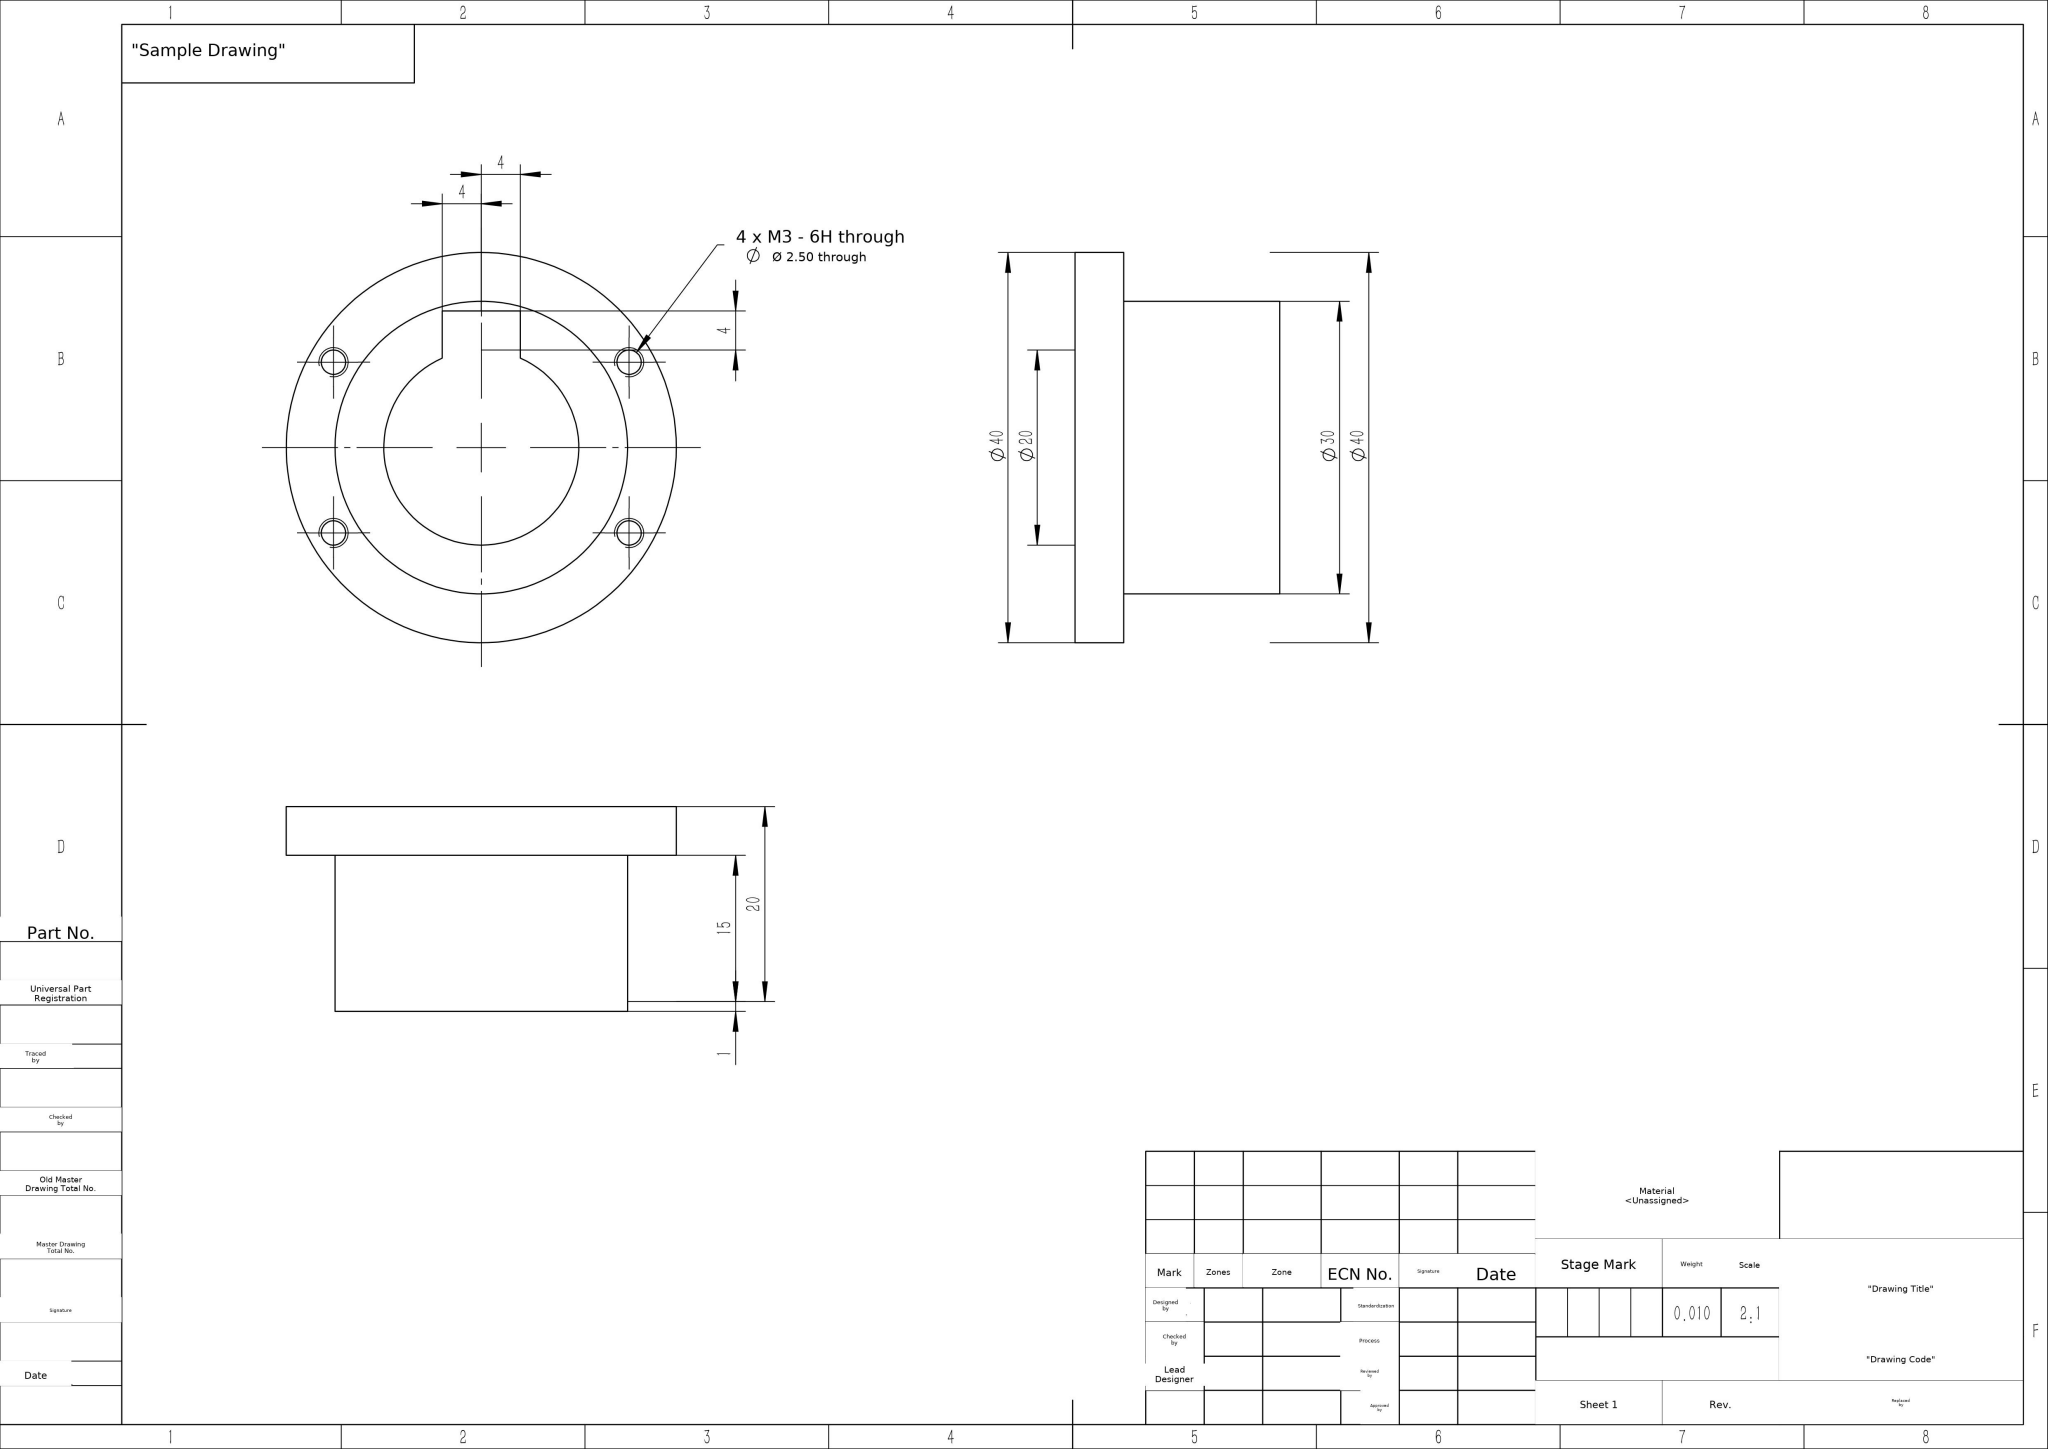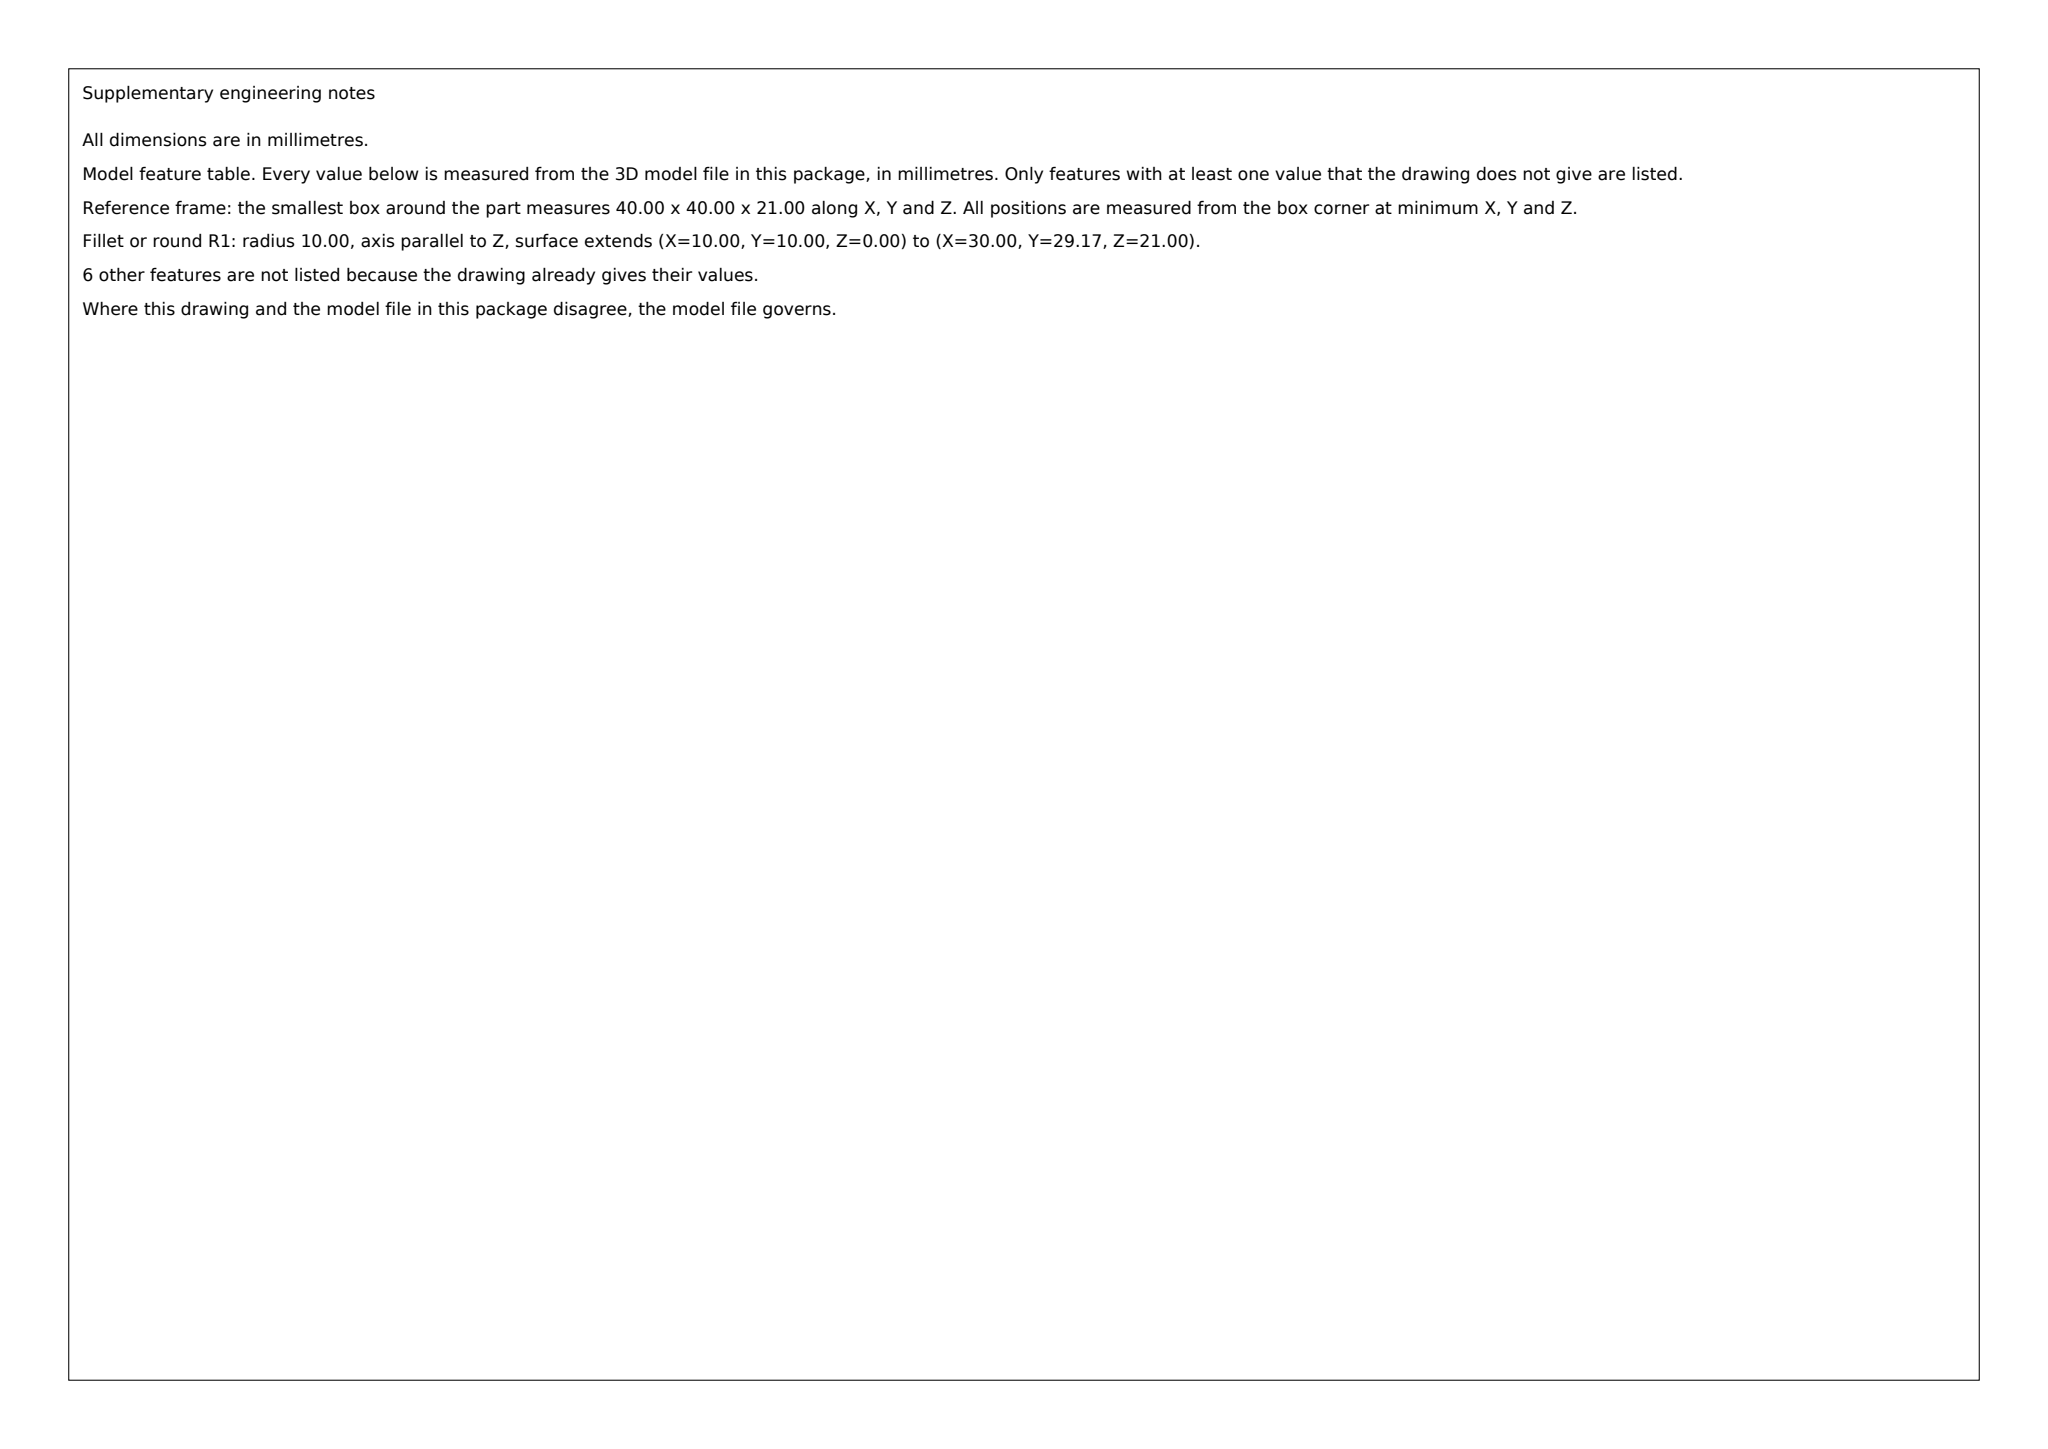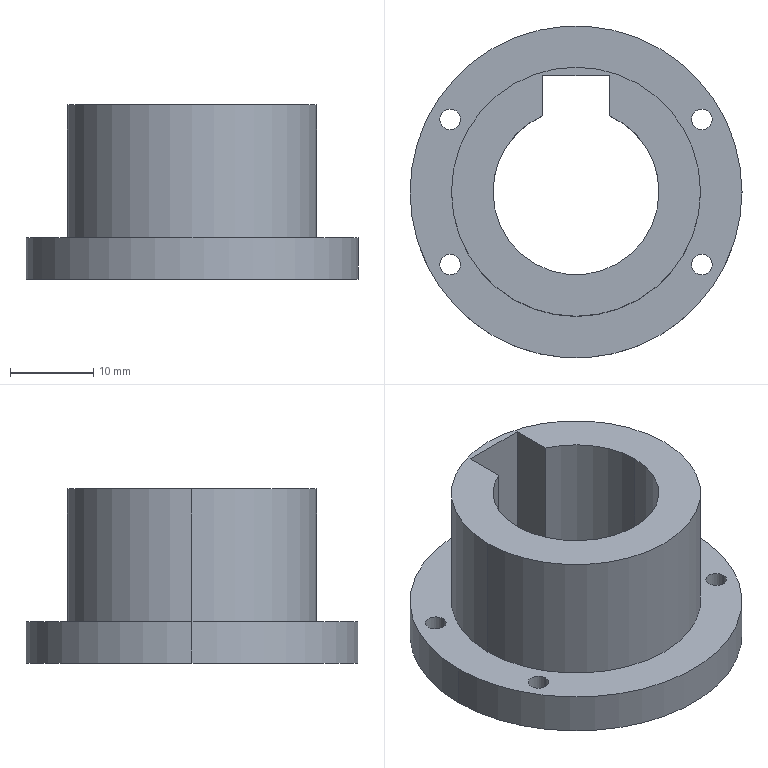Part | SolidWorks | mm | 1 solid | 21 faces | box 40 x 40 x 21 mm | volume 10179 mm3 | cylinder 15 | plane 6 | commonest cylinder face diameters 2.5 x8 20 x3 30 x2 40 x2
build123d program:
from build123d import *

# Parameters (mm, degrees)
SKETCH1_R           = 20
SKETCH1_R_2         = 10
BOSS_EXTRUDE1_DEPTH = 20
CUT_EXTRUDE1_START  = -20
CUT_EXTRUDE1_DEPTH  = 20
CUT_EXTRUDE3_START  = -15
SKETCH4_R           = 20
SKETCH4_R_2         = 15
CUT_EXTRUDE3_DEPTH  = 15
M3_TAPPED_HOLE1_D   = 2.5
SKETCH7_R           = 15
BOSS_EXTRUDE2_DEPTH = 1


with BuildPart() as part:
    # Sketch1 → Boss-Extrude1 (new body)
    with BuildSketch(Plane.XY):
        Circle(SKETCH1_R)
        Circle(SKETCH1_R_2, mode=Mode.SUBTRACT)
    extrude(amount=BOSS_EXTRUDE1_DEPTH)

    # Sketch3 → Cut-Extrude1 (cut)
    with BuildSketch(Plane.XY.offset(20).offset(CUT_EXTRUDE1_START)):
        with BuildLine():
            ThreePointArc((-4, 9.165), (-2.043, 9.789), (0, 10))
            Line((0, 10), (0, 14))
            Line((0, 14), (-4, 14))
            Line((-4, 14), (-4, 9.165))
        make_face()
        with BuildLine():
            Line((0, 14), (0, 10))
            ThreePointArc((0, 10), (2.043, 9.789), (4, 9.165))
            Line((4, 9.165), (4, 14))
            Line((4, 14), (0, 14))
        make_face()
    extrude(amount=CUT_EXTRUDE1_DEPTH, mode=Mode.SUBTRACT)

    # Sketch4 → Cut-Extrude3 (cut)
    with BuildSketch(Plane.XY.offset(20).offset(CUT_EXTRUDE3_START)):
        Circle(SKETCH4_R)
        Circle(SKETCH4_R_2, mode=Mode.SUBTRACT)
    extrude(amount=CUT_EXTRUDE3_DEPTH, mode=Mode.SUBTRACT)

    # M3 Tapped Hole1 (through all)
    with Locations(Plane(origin=(15.155, 8.75, 0), x_dir=(-1, 0, 0), z_dir=(0, 0, -1))):
        with Locations((0, 0), (30.311, 0), (30.311, -17.5), (0, -17.5)):
            Hole(M3_TAPPED_HOLE1_D / 2)

    # Sketch7 → Boss-Extrude2 (add)
    with BuildSketch(Plane.XY.offset(20)):
        Circle(SKETCH7_R)
        with BuildLine():
            Line((-4, 9.165), (-4, 14))
            Line((-4, 14), (4, 14))
            Line((4, 14), (4, 9.165))
            ThreePointArc((4, 9.165), (0, -10), (-4, 9.165))
        make_face(mode=Mode.SUBTRACT)
    extrude(amount=BOSS_EXTRUDE2_DEPTH)


solid = part.part
STEP:
#1=CARTESIAN_POINT('',(13.905,8.75,5.));
#2=VERTEX_POINT('',#1);
#3=CARTESIAN_POINT('',(16.405,8.75,5.));
#4=VERTEX_POINT('',#3);
#5=CARTESIAN_POINT('',(15.155,8.75,5.));
#6=DIRECTION('',(0.,0.,1.));
#7=DIRECTION('',(1.,0.,0.));
#8=AXIS2_PLACEMENT_3D('',#5,#6,#7);
#9=CIRCLE('',#8,1.25);
#10=EDGE_CURVE('',#2,#4,#9,.T.);
#11=ORIENTED_EDGE('',*,*,#10,.T.);
#12=CARTESIAN_POINT('',(16.405,8.75,-0.));
#13=VERTEX_POINT('',#12);
#14=CARTESIAN_POINT('',(16.405,8.75,0.));
#15=DIRECTION('',(0.,0.,-1.));
#16=VECTOR('',#15,1000.);
#17=LINE('',#14,#16);
#18=EDGE_CURVE('',#4,#13,#17,.T.);
#19=ORIENTED_EDGE('',*,*,#18,.T.);
#20=CARTESIAN_POINT('',(13.905,8.75,-0.));
#21=VERTEX_POINT('',#20);
#22=CARTESIAN_POINT('',(15.155,8.75,-0.));
#23=DIRECTION('',(0.,0.,-1.));
#24=DIRECTION('',(-1.,0.,0.));
#25=AXIS2_PLACEMENT_3D('',#22,#23,#24);
#26=CIRCLE('',#25,1.25);
#27=EDGE_CURVE('',#13,#21,#26,.T.);
#28=ORIENTED_EDGE('',*,*,#27,.T.);
#29=CARTESIAN_POINT('',(13.905,8.75,0.));
#30=DIRECTION('',(0.,0.,-1.));
#31=VECTOR('',#30,1000.);
#32=LINE('',#29,#31);
#33=EDGE_CURVE('',#2,#21,#32,.T.);
#34=ORIENTED_EDGE('',*,*,#33,.F.);
#35=EDGE_LOOP('',(#11,#19,#28,#34));
#36=FACE_OUTER_BOUND('',#35,.T.);
#37=CARTESIAN_POINT('',(15.155,8.75,0.));
#38=DIRECTION('',(0.,0.,-1.));
#39=DIRECTION('',(-1.,0.,0.));
#40=AXIS2_PLACEMENT_3D('',#37,#38,#39);
#41=CYLINDRICAL_SURFACE('',#40,1.25);
#42=ADVANCED_FACE('',(#36),#41,.F.);
#43=CARTESIAN_POINT('',(-16.405,8.75,5.));
#44=VERTEX_POINT('',#43);
#45=CARTESIAN_POINT('',(-13.905,8.75,5.));
#46=VERTEX_POINT('',#45);
#47=CARTESIAN_POINT('',(-15.155,8.75,5.));
#48=DIRECTION('',(0.,0.,1.));
#49=DIRECTION('',(1.,0.,0.));
#50=AXIS2_PLACEMENT_3D('',#47,#48,#49);
#51=CIRCLE('',#50,1.25);
#52=EDGE_CURVE('',#44,#46,#51,.T.);
#53=ORIENTED_EDGE('',*,*,#52,.T.);
#54=CARTESIAN_POINT('',(-13.905,8.75,-0.));
#55=VERTEX_POINT('',#54);
#56=CARTESIAN_POINT('',(-13.905,8.75,0.));
#57=DIRECTION('',(0.,0.,-1.));
#58=VECTOR('',#57,1000.);
#59=LINE('',#56,#58);
#60=EDGE_CURVE('',#46,#55,#59,.T.);
#61=ORIENTED_EDGE('',*,*,#60,.T.);
#62=CARTESIAN_POINT('',(-16.405,8.75,-0.));
#63=VERTEX_POINT('',#62);
#64=CARTESIAN_POINT('',(-15.155,8.75,-0.));
#65=DIRECTION('',(0.,0.,-1.));
#66=DIRECTION('',(-1.,0.,0.));
#67=AXIS2_PLACEMENT_3D('',#64,#65,#66);
#68=CIRCLE('',#67,1.25);
#69=EDGE_CURVE('',#55,#63,#68,.T.);
#70=ORIENTED_EDGE('',*,*,#69,.T.);
#71=CARTESIAN_POINT('',(-16.405,8.75,0.));
#72=DIRECTION('',(0.,0.,-1.));
#73=VECTOR('',#72,1000.);
#74=LINE('',#71,#73);
#75=EDGE_CURVE('',#44,#63,#74,.T.);
#76=ORIENTED_EDGE('',*,*,#75,.F.);
#77=EDGE_LOOP('',(#53,#61,#70,#76));
#78=FACE_OUTER_BOUND('',#77,.T.);
#79=CARTESIAN_POINT('',(-15.155,8.75,0.));
#80=DIRECTION('',(0.,0.,-1.));
#81=DIRECTION('',(-1.,0.,0.));
#82=AXIS2_PLACEMENT_3D('',#79,#80,#81);
#83=CYLINDRICAL_SURFACE('',#82,1.25);
#84=ADVANCED_FACE('',(#78),#83,.F.);
#85=CARTESIAN_POINT('',(-16.405,-8.75,5.));
#86=VERTEX_POINT('',#85);
#87=CARTESIAN_POINT('',(-13.905,-8.75,5.));
#88=VERTEX_POINT('',#87);
#89=CARTESIAN_POINT('',(-15.155,-8.75,5.));
#90=DIRECTION('',(0.,0.,1.));
#91=DIRECTION('',(1.,0.,0.));
#92=AXIS2_PLACEMENT_3D('',#89,#90,#91);
#93=CIRCLE('',#92,1.25);
#94=EDGE_CURVE('',#86,#88,#93,.T.);
#95=ORIENTED_EDGE('',*,*,#94,.T.);
#96=CARTESIAN_POINT('',(-13.905,-8.75,-0.));
#97=VERTEX_POINT('',#96);
#98=CARTESIAN_POINT('',(-13.905,-8.75,0.));
#99=DIRECTION('',(0.,0.,-1.));
#100=VECTOR('',#99,1000.);
#101=LINE('',#98,#100);
#102=EDGE_CURVE('',#88,#97,#101,.T.);
#103=ORIENTED_EDGE('',*,*,#102,.T.);
#104=CARTESIAN_POINT('',(-16.405,-8.75,-0.));
#105=VERTEX_POINT('',#104);
#106=CARTESIAN_POINT('',(-15.155,-8.75,-0.));
#107=DIRECTION('',(0.,0.,-1.));
#108=DIRECTION('',(-1.,0.,0.));
#109=AXIS2_PLACEMENT_3D('',#106,#107,#108);
#110=CIRCLE('',#109,1.25);
#111=EDGE_CURVE('',#97,#105,#110,.T.);
#112=ORIENTED_EDGE('',*,*,#111,.T.);
#113=CARTESIAN_POINT('',(-16.405,-8.75,0.));
#114=DIRECTION('',(0.,0.,-1.));
#115=VECTOR('',#114,1000.);
#116=LINE('',#113,#115);
#117=EDGE_CURVE('',#86,#105,#116,.T.);
#118=ORIENTED_EDGE('',*,*,#117,.F.);
#119=EDGE_LOOP('',(#95,#103,#112,#118));
#120=FACE_OUTER_BOUND('',#119,.T.);
#121=CARTESIAN_POINT('',(-15.155,-8.75,0.));
#122=DIRECTION('',(0.,0.,-1.));
#123=DIRECTION('',(-1.,0.,0.));
#124=AXIS2_PLACEMENT_3D('',#121,#122,#123);
#125=CYLINDRICAL_SURFACE('',#124,1.25);
#126=ADVANCED_FACE('',(#120),#125,.F.);
#127=CARTESIAN_POINT('',(13.905,-8.75,5.));
#128=VERTEX_POINT('',#127);
#129=CARTESIAN_POINT('',(16.405,-8.75,5.));
#130=VERTEX_POINT('',#129);
#131=CARTESIAN_POINT('',(15.155,-8.75,5.));
#132=DIRECTION('',(0.,0.,1.));
#133=DIRECTION('',(1.,0.,0.));
#134=AXIS2_PLACEMENT_3D('',#131,#132,#133);
#135=CIRCLE('',#134,1.25);
#136=EDGE_CURVE('',#128,#130,#135,.T.);
#137=ORIENTED_EDGE('',*,*,#136,.T.);
#138=CARTESIAN_POINT('',(16.405,-8.75,-0.));
#139=VERTEX_POINT('',#138);
#140=CARTESIAN_POINT('',(16.405,-8.75,0.));
#141=DIRECTION('',(0.,0.,-1.));
#142=VECTOR('',#141,1000.);
#143=LINE('',#140,#142);
#144=EDGE_CURVE('',#130,#139,#143,.T.);
#145=ORIENTED_EDGE('',*,*,#144,.T.);
#146=CARTESIAN_POINT('',(13.905,-8.75,-0.));
#147=VERTEX_POINT('',#146);
#148=CARTESIAN_POINT('',(15.155,-8.75,-0.));
#149=DIRECTION('',(0.,0.,-1.));
#150=DIRECTION('',(-1.,0.,0.));
#151=AXIS2_PLACEMENT_3D('',#148,#149,#150);
#152=CIRCLE('',#151,1.25);
#153=EDGE_CURVE('',#139,#147,#152,.T.);
#154=ORIENTED_EDGE('',*,*,#153,.T.);
#155=CARTESIAN_POINT('',(13.905,-8.75,0.));
#156=DIRECTION('',(0.,0.,-1.));
#157=VECTOR('',#156,1000.);
#158=LINE('',#155,#157);
#159=EDGE_CURVE('',#128,#147,#158,.T.);
#160=ORIENTED_EDGE('',*,*,#159,.F.);
#161=EDGE_LOOP('',(#137,#145,#154,#160));
#162=FACE_OUTER_BOUND('',#161,.T.);
#163=CARTESIAN_POINT('',(15.155,-8.75,0.));
#164=DIRECTION('',(0.,0.,-1.));
#165=DIRECTION('',(-1.,0.,0.));
#166=AXIS2_PLACEMENT_3D('',#163,#164,#165);
#167=CYLINDRICAL_SURFACE('',#166,1.25);
#168=ADVANCED_FACE('',(#162),#167,.F.);
#169=CARTESIAN_POINT('',(15.,0.,5.));
#170=VERTEX_POINT('',#169);
#171=CARTESIAN_POINT('',(-15.,0.,5.));
#172=VERTEX_POINT('',#171);
#173=CARTESIAN_POINT('',(0.,0.,5.));
#174=DIRECTION('',(0.,0.,1.));
#175=DIRECTION('',(1.,0.,0.));
#176=AXIS2_PLACEMENT_3D('',#173,#174,#175);
#177=CIRCLE('',#176,15.);
#178=EDGE_CURVE('',#170,#172,#177,.T.);
#179=ORIENTED_EDGE('',*,*,#178,.T.);
#180=CARTESIAN_POINT('',(-15.,0.,21.));
#181=VERTEX_POINT('',#180);
#182=CARTESIAN_POINT('',(-15.,0.,5.));
#183=DIRECTION('',(0.,0.,1.));
#184=VECTOR('',#183,1000.);
#185=LINE('',#182,#184);
#186=EDGE_CURVE('',#172,#181,#185,.T.);
#187=ORIENTED_EDGE('',*,*,#186,.T.);
#188=CARTESIAN_POINT('',(15.,0.,21.));
#189=VERTEX_POINT('',#188);
#190=CARTESIAN_POINT('',(0.,0.,21.));
#191=DIRECTION('',(0.,0.,1.));
#192=DIRECTION('',(1.,0.,0.));
#193=AXIS2_PLACEMENT_3D('',#190,#191,#192);
#194=CIRCLE('',#193,15.);
#195=EDGE_CURVE('',#189,#181,#194,.T.);
#196=ORIENTED_EDGE('',*,*,#195,.F.);
#197=CARTESIAN_POINT('',(15.,0.,5.));
#198=DIRECTION('',(0.,0.,1.));
#199=VECTOR('',#198,1000.);
#200=LINE('',#197,#199);
#201=EDGE_CURVE('',#170,#189,#200,.T.);
#202=ORIENTED_EDGE('',*,*,#201,.F.);
#203=EDGE_LOOP('',(#179,#187,#196,#202));
#204=FACE_OUTER_BOUND('',#203,.T.);
#205=CARTESIAN_POINT('',(0.,0.,5.));
#206=DIRECTION('',(0.,0.,1.));
#207=DIRECTION('',(1.,0.,0.));
#208=AXIS2_PLACEMENT_3D('',#205,#206,#207);
#209=CYLINDRICAL_SURFACE('',#208,15.);
#210=ADVANCED_FACE('',(#204),#209,.T.);
#211=CARTESIAN_POINT('',(-10.,0.,21.));
#212=VERTEX_POINT('',#211);
#213=CARTESIAN_POINT('',(10.,0.,21.));
#214=VERTEX_POINT('',#213);
#215=CARTESIAN_POINT('',(0.,0.,21.));
#216=DIRECTION('',(0.,0.,1.));
#217=DIRECTION('',(1.,0.,0.));
#218=AXIS2_PLACEMENT_3D('',#215,#216,#217);
#219=CIRCLE('',#218,10.);
#220=EDGE_CURVE('',#212,#214,#219,.T.);
#221=ORIENTED_EDGE('',*,*,#220,.T.);
#222=CARTESIAN_POINT('',(10.,0.,0.));
#223=VERTEX_POINT('',#222);
#224=CARTESIAN_POINT('',(10.,0.,20.));
#225=DIRECTION('',(0.,0.,-1.));
#226=VECTOR('',#225,1000.);
#227=LINE('',#224,#226);
#228=EDGE_CURVE('',#214,#223,#227,.T.);
#229=ORIENTED_EDGE('',*,*,#228,.T.);
#230=CARTESIAN_POINT('',(-10.,0.,0.));
#231=VERTEX_POINT('',#230);
#232=CARTESIAN_POINT('',(0.,0.,0.));
#233=DIRECTION('',(0.,0.,1.));
#234=DIRECTION('',(1.,0.,0.));
#235=AXIS2_PLACEMENT_3D('',#232,#233,#234);
#236=CIRCLE('',#235,10.);
#237=EDGE_CURVE('',#231,#223,#236,.T.);
#238=ORIENTED_EDGE('',*,*,#237,.F.);
#239=CARTESIAN_POINT('',(-10.,0.,20.));
#240=DIRECTION('',(0.,0.,-1.));
#241=VECTOR('',#240,1000.);
#242=LINE('',#239,#241);
#243=EDGE_CURVE('',#212,#231,#242,.T.);
#244=ORIENTED_EDGE('',*,*,#243,.F.);
#245=EDGE_LOOP('',(#221,#229,#238,#244));
#246=FACE_OUTER_BOUND('',#245,.T.);
#247=CARTESIAN_POINT('',(0.,0.,20.));
#248=DIRECTION('',(0.,0.,-1.));
#249=DIRECTION('',(-1.,0.,0.));
#250=AXIS2_PLACEMENT_3D('',#247,#248,#249);
#251=CYLINDRICAL_SURFACE('',#250,10.);
#252=ADVANCED_FACE('',(#246),#251,.F.);
#253=CARTESIAN_POINT('',(-4.,9.165,21.));
#254=VERTEX_POINT('',#253);
#255=CARTESIAN_POINT('',(0.,0.,21.));
#256=DIRECTION('',(0.,0.,1.));
#257=DIRECTION('',(1.,0.,0.));
#258=AXIS2_PLACEMENT_3D('',#255,#256,#257);
#259=CIRCLE('',#258,10.);
#260=EDGE_CURVE('',#254,#212,#259,.T.);
#261=ORIENTED_EDGE('',*,*,#260,.T.);
#262=ORIENTED_EDGE('',*,*,#243,.T.);
#263=CARTESIAN_POINT('',(-4.,9.165,0.));
#264=VERTEX_POINT('',#263);
#265=CARTESIAN_POINT('',(0.,0.,0.));
#266=DIRECTION('',(0.,0.,1.));
#267=DIRECTION('',(1.,0.,0.));
#268=AXIS2_PLACEMENT_3D('',#265,#266,#267);
#269=CIRCLE('',#268,10.);
#270=EDGE_CURVE('',#264,#231,#269,.T.);
#271=ORIENTED_EDGE('',*,*,#270,.F.);
#272=CARTESIAN_POINT('',(-4.,9.165,0.));
#273=DIRECTION('',(0.,0.,1.));
#274=VECTOR('',#273,1000.);
#275=LINE('',#272,#274);
#276=EDGE_CURVE('',#264,#254,#275,.T.);
#277=ORIENTED_EDGE('',*,*,#276,.T.);
#278=EDGE_LOOP('',(#261,#262,#271,#277));
#279=FACE_OUTER_BOUND('',#278,.T.);
#280=CARTESIAN_POINT('',(0.,0.,20.));
#281=DIRECTION('',(0.,0.,-1.));
#282=DIRECTION('',(-1.,0.,0.));
#283=AXIS2_PLACEMENT_3D('',#280,#281,#282);
#284=CYLINDRICAL_SURFACE('',#283,10.);
#285=ADVANCED_FACE('',(#279),#284,.F.);
#286=CARTESIAN_POINT('',(20.,0.,5.));
#287=VERTEX_POINT('',#286);
#288=CARTESIAN_POINT('',(-20.,0.,5.));
#289=VERTEX_POINT('',#288);
#290=CARTESIAN_POINT('',(0.,0.,5.));
#291=DIRECTION('',(0.,0.,1.));
#292=DIRECTION('',(1.,0.,0.));
#293=AXIS2_PLACEMENT_3D('',#290,#291,#292);
#294=CIRCLE('',#293,20.);
#295=EDGE_CURVE('',#287,#289,#294,.T.);
#296=ORIENTED_EDGE('',*,*,#295,.F.);
#297=CARTESIAN_POINT('',(20.,0.,0.));
#298=VERTEX_POINT('',#297);
#299=CARTESIAN_POINT('',(20.,0.,20.));
#300=DIRECTION('',(0.,0.,-1.));
#301=VECTOR('',#300,1000.);
#302=LINE('',#299,#301);
#303=EDGE_CURVE('',#287,#298,#302,.T.);
#304=ORIENTED_EDGE('',*,*,#303,.T.);
#305=CARTESIAN_POINT('',(-20.,0.,0.));
#306=VERTEX_POINT('',#305);
#307=CARTESIAN_POINT('',(0.,0.,0.));
#308=DIRECTION('',(0.,0.,1.));
#309=DIRECTION('',(1.,0.,0.));
#310=AXIS2_PLACEMENT_3D('',#307,#308,#309);
#311=CIRCLE('',#310,20.);
#312=EDGE_CURVE('',#298,#306,#311,.T.);
#313=ORIENTED_EDGE('',*,*,#312,.T.);
#314=CARTESIAN_POINT('',(-20.,0.,20.));
#315=DIRECTION('',(0.,0.,-1.));
#316=VECTOR('',#315,1000.);
#317=LINE('',#314,#316);
#318=EDGE_CURVE('',#289,#306,#317,.T.);
#319=ORIENTED_EDGE('',*,*,#318,.F.);
#320=EDGE_LOOP('',(#296,#304,#313,#319));
#321=FACE_OUTER_BOUND('',#320,.T.);
#322=CARTESIAN_POINT('',(0.,0.,20.));
#323=DIRECTION('',(0.,0.,-1.));
#324=DIRECTION('',(-1.,0.,0.));
#325=AXIS2_PLACEMENT_3D('',#322,#323,#324);
#326=CYLINDRICAL_SURFACE('',#325,20.);
#327=ADVANCED_FACE('',(#321),#326,.T.);
#328=CARTESIAN_POINT('',(4.,14.,0.));
#329=VERTEX_POINT('',#328);
#330=CARTESIAN_POINT('',(4.,9.165,0.));
#331=VERTEX_POINT('',#330);
#332=CARTESIAN_POINT('',(4.,0.,0.));
#333=DIRECTION('',(0.,-1.,0.));
#334=VECTOR('',#333,1000.);
#335=LINE('',#332,#334);
#336=EDGE_CURVE('',#329,#331,#335,.T.);
#337=ORIENTED_EDGE('',*,*,#336,.F.);
#338=CARTESIAN_POINT('',(-4.,14.,0.));
#339=VERTEX_POINT('',#338);
#340=CARTESIAN_POINT('',(0.,14.,0.));
#341=DIRECTION('',(-1.,0.,0.));
#342=VECTOR('',#341,1000.);
#343=LINE('',#340,#342);
#344=EDGE_CURVE('',#329,#339,#343,.T.);
#345=ORIENTED_EDGE('',*,*,#344,.T.);
#346=CARTESIAN_POINT('',(-4.,0.,0.));
#347=DIRECTION('',(0.,-1.,0.));
#348=VECTOR('',#347,1000.);
#349=LINE('',#346,#348);
#350=EDGE_CURVE('',#339,#264,#349,.T.);
#351=ORIENTED_EDGE('',*,*,#350,.T.);
#352=ORIENTED_EDGE('',*,*,#270,.T.);
#353=ORIENTED_EDGE('',*,*,#237,.T.);
#354=CARTESIAN_POINT('',(0.,0.,0.));
#355=DIRECTION('',(0.,0.,1.));
#356=DIRECTION('',(1.,0.,0.));
#357=AXIS2_PLACEMENT_3D('',#354,#355,#356);
#358=CIRCLE('',#357,10.);
#359=EDGE_CURVE('',#223,#331,#358,.T.);
#360=ORIENTED_EDGE('',*,*,#359,.T.);
#361=EDGE_LOOP('',(#337,#345,#351,#352,#353,#360));
#362=FACE_BOUND('',#361,.T.);
#363=CARTESIAN_POINT('',(0.,0.,0.));
#364=DIRECTION('',(0.,0.,1.));
#365=DIRECTION('',(1.,0.,0.));
#366=AXIS2_PLACEMENT_3D('',#363,#364,#365);
#367=CIRCLE('',#366,20.);
#368=EDGE_CURVE('',#306,#298,#367,.T.);
#369=ORIENTED_EDGE('',*,*,#368,.F.);
#370=ORIENTED_EDGE('',*,*,#312,.F.);
#371=EDGE_LOOP('',(#369,#370));
#372=FACE_OUTER_BOUND('',#371,.T.);
#373=CARTESIAN_POINT('',(15.155,-8.75,-0.));
#374=DIRECTION('',(0.,0.,-1.));
#375=DIRECTION('',(-1.,0.,0.));
#376=AXIS2_PLACEMENT_3D('',#373,#374,#375);
#377=CIRCLE('',#376,1.25);
#378=EDGE_CURVE('',#147,#139,#377,.T.);
#379=ORIENTED_EDGE('',*,*,#378,.F.);
#380=ORIENTED_EDGE('',*,*,#153,.F.);
#381=EDGE_LOOP('',(#379,#380));
#382=FACE_BOUND('',#381,.T.);
#383=CARTESIAN_POINT('',(-15.155,-8.75,-0.));
#384=DIRECTION('',(0.,0.,-1.));
#385=DIRECTION('',(-1.,0.,0.));
#386=AXIS2_PLACEMENT_3D('',#383,#384,#385);
#387=CIRCLE('',#386,1.25);
#388=EDGE_CURVE('',#105,#97,#387,.T.);
#389=ORIENTED_EDGE('',*,*,#388,.F.);
#390=ORIENTED_EDGE('',*,*,#111,.F.);
#391=EDGE_LOOP('',(#389,#390));
#392=FACE_BOUND('',#391,.T.);
#393=CARTESIAN_POINT('',(-15.155,8.75,-0.));
#394=DIRECTION('',(0.,0.,-1.));
#395=DIRECTION('',(-1.,0.,0.));
#396=AXIS2_PLACEMENT_3D('',#393,#394,#395);
#397=CIRCLE('',#396,1.25);
#398=EDGE_CURVE('',#63,#55,#397,.T.);
#399=ORIENTED_EDGE('',*,*,#398,.F.);
#400=ORIENTED_EDGE('',*,*,#69,.F.);
#401=EDGE_LOOP('',(#399,#400));
#402=FACE_BOUND('',#401,.T.);
#403=CARTESIAN_POINT('',(15.155,8.75,-0.));
#404=DIRECTION('',(0.,0.,-1.));
#405=DIRECTION('',(-1.,0.,0.));
#406=AXIS2_PLACEMENT_3D('',#403,#404,#405);
#407=CIRCLE('',#406,1.25);
#408=EDGE_CURVE('',#21,#13,#407,.T.);
#409=ORIENTED_EDGE('',*,*,#408,.F.);
#410=ORIENTED_EDGE('',*,*,#27,.F.);
#411=EDGE_LOOP('',(#409,#410));
#412=FACE_BOUND('',#411,.T.);
#413=CARTESIAN_POINT('',(0.,0.,0.));
#414=DIRECTION('',(0.,0.,1.));
#415=DIRECTION('',(1.,0.,0.));
#416=AXIS2_PLACEMENT_3D('',#413,#414,#415);
#417=PLANE('',#416);
#418=ADVANCED_FACE('',(#362,#372,#382,#392,#402,#412),#417,.F.);
#419=ORIENTED_EDGE('',*,*,#303,.F.);
#420=CARTESIAN_POINT('',(0.,0.,5.));
#421=DIRECTION('',(0.,0.,1.));
#422=DIRECTION('',(1.,0.,0.));
#423=AXIS2_PLACEMENT_3D('',#420,#421,#422);
#424=CIRCLE('',#423,20.);
#425=EDGE_CURVE('',#289,#287,#424,.T.);
#426=ORIENTED_EDGE('',*,*,#425,.F.);
#427=ORIENTED_EDGE('',*,*,#318,.T.);
#428=ORIENTED_EDGE('',*,*,#368,.T.);
#429=EDGE_LOOP('',(#419,#426,#427,#428));
#430=FACE_OUTER_BOUND('',#429,.T.);
#431=CARTESIAN_POINT('',(0.,0.,20.));
#432=DIRECTION('',(0.,0.,-1.));
#433=DIRECTION('',(-1.,0.,0.));
#434=AXIS2_PLACEMENT_3D('',#431,#432,#433);
#435=CYLINDRICAL_SURFACE('',#434,20.);
#436=ADVANCED_FACE('',(#430),#435,.T.);
#437=ORIENTED_EDGE('',*,*,#228,.F.);
#438=CARTESIAN_POINT('',(4.,9.165,21.));
#439=VERTEX_POINT('',#438);
#440=CARTESIAN_POINT('',(0.,0.,21.));
#441=DIRECTION('',(0.,0.,1.));
#442=DIRECTION('',(1.,0.,0.));
#443=AXIS2_PLACEMENT_3D('',#440,#441,#442);
#444=CIRCLE('',#443,10.);
#445=EDGE_CURVE('',#214,#439,#444,.T.);
#446=ORIENTED_EDGE('',*,*,#445,.T.);
#447=CARTESIAN_POINT('',(4.,9.165,0.));
#448=DIRECTION('',(0.,0.,1.));
#449=VECTOR('',#448,1000.);
#450=LINE('',#447,#449);
#451=EDGE_CURVE('',#331,#439,#450,.T.);
#452=ORIENTED_EDGE('',*,*,#451,.F.);
#453=ORIENTED_EDGE('',*,*,#359,.F.);
#454=EDGE_LOOP('',(#437,#446,#452,#453));
#455=FACE_OUTER_BOUND('',#454,.T.);
#456=CARTESIAN_POINT('',(0.,0.,20.));
#457=DIRECTION('',(0.,0.,-1.));
#458=DIRECTION('',(-1.,0.,0.));
#459=AXIS2_PLACEMENT_3D('',#456,#457,#458);
#460=CYLINDRICAL_SURFACE('',#459,10.);
#461=ADVANCED_FACE('',(#455),#460,.F.);
#462=CARTESIAN_POINT('',(4.,14.,21.));
#463=VERTEX_POINT('',#462);
#464=CARTESIAN_POINT('',(4.,14.,0.));
#465=DIRECTION('',(0.,0.,1.));
#466=VECTOR('',#465,1000.);
#467=LINE('',#464,#466);
#468=EDGE_CURVE('',#329,#463,#467,.T.);
#469=ORIENTED_EDGE('',*,*,#468,.T.);
#470=CARTESIAN_POINT('',(-4.,14.,21.));
#471=VERTEX_POINT('',#470);
#472=CARTESIAN_POINT('',(-4.,14.,21.));
#473=DIRECTION('',(-1.,0.,0.));
#474=VECTOR('',#473,1000.);
#475=LINE('',#472,#474);
#476=EDGE_CURVE('',#463,#471,#475,.T.);
#477=ORIENTED_EDGE('',*,*,#476,.T.);
#478=CARTESIAN_POINT('',(-4.,14.,0.));
#479=DIRECTION('',(0.,0.,1.));
#480=VECTOR('',#479,1000.);
#481=LINE('',#478,#480);
#482=EDGE_CURVE('',#339,#471,#481,.T.);
#483=ORIENTED_EDGE('',*,*,#482,.F.);
#484=ORIENTED_EDGE('',*,*,#344,.F.);
#485=EDGE_LOOP('',(#469,#477,#483,#484));
#486=FACE_OUTER_BOUND('',#485,.T.);
#487=CARTESIAN_POINT('',(0.,14.,0.));
#488=DIRECTION('',(0.,1.,0.));
#489=DIRECTION('',(0.,0.,1.));
#490=AXIS2_PLACEMENT_3D('',#487,#488,#489);
#491=PLANE('',#490);
#492=ADVANCED_FACE('',(#486),#491,.F.);
#493=ORIENTED_EDGE('',*,*,#451,.T.);
#494=CARTESIAN_POINT('',(4.,14.,21.));
#495=DIRECTION('',(0.,1.,0.));
#496=VECTOR('',#495,1000.);
#497=LINE('',#494,#496);
#498=EDGE_CURVE('',#439,#463,#497,.T.);
#499=ORIENTED_EDGE('',*,*,#498,.T.);
#500=ORIENTED_EDGE('',*,*,#468,.F.);
#501=ORIENTED_EDGE('',*,*,#336,.T.);
#502=EDGE_LOOP('',(#493,#499,#500,#501));
#503=FACE_OUTER_BOUND('',#502,.T.);
#504=CARTESIAN_POINT('',(4.,0.,0.));
#505=DIRECTION('',(-1.,0.,0.));
#506=DIRECTION('',(0.,0.,1.));
#507=AXIS2_PLACEMENT_3D('',#504,#505,#506);
#508=PLANE('',#507);
#509=ADVANCED_FACE('',(#503),#508,.T.);
#510=ORIENTED_EDGE('',*,*,#482,.T.);
#511=CARTESIAN_POINT('',(-4.,9.165,21.));
#512=DIRECTION('',(0.,-1.,0.));
#513=VECTOR('',#512,1000.);
#514=LINE('',#511,#513);
#515=EDGE_CURVE('',#471,#254,#514,.T.);
#516=ORIENTED_EDGE('',*,*,#515,.T.);
#517=ORIENTED_EDGE('',*,*,#276,.F.);
#518=ORIENTED_EDGE('',*,*,#350,.F.);
#519=EDGE_LOOP('',(#510,#516,#517,#518));
#520=FACE_OUTER_BOUND('',#519,.T.);
#521=CARTESIAN_POINT('',(-4.,0.,0.));
#522=DIRECTION('',(-1.,0.,0.));
#523=DIRECTION('',(0.,0.,1.));
#524=AXIS2_PLACEMENT_3D('',#521,#522,#523);
#525=PLANE('',#524);
#526=ADVANCED_FACE('',(#520),#525,.F.);
#527=ORIENTED_EDGE('',*,*,#10,.F.);
#528=CARTESIAN_POINT('',(15.155,8.75,5.));
#529=DIRECTION('',(0.,0.,1.));
#530=DIRECTION('',(1.,0.,0.));
#531=AXIS2_PLACEMENT_3D('',#528,#529,#530);
#532=CIRCLE('',#531,1.25);
#533=EDGE_CURVE('',#4,#2,#532,.T.);
#534=ORIENTED_EDGE('',*,*,#533,.F.);
#535=EDGE_LOOP('',(#527,#534));
#536=FACE_BOUND('',#535,.T.);
#537=ORIENTED_EDGE('',*,*,#52,.F.);
#538=CARTESIAN_POINT('',(-15.155,8.75,5.));
#539=DIRECTION('',(0.,0.,1.));
#540=DIRECTION('',(1.,0.,0.));
#541=AXIS2_PLACEMENT_3D('',#538,#539,#540);
#542=CIRCLE('',#541,1.25);
#543=EDGE_CURVE('',#46,#44,#542,.T.);
#544=ORIENTED_EDGE('',*,*,#543,.F.);
#545=EDGE_LOOP('',(#537,#544));
#546=FACE_BOUND('',#545,.T.);
#547=ORIENTED_EDGE('',*,*,#94,.F.);
#548=CARTESIAN_POINT('',(-15.155,-8.75,5.));
#549=DIRECTION('',(0.,0.,1.));
#550=DIRECTION('',(1.,0.,0.));
#551=AXIS2_PLACEMENT_3D('',#548,#549,#550);
#552=CIRCLE('',#551,1.25);
#553=EDGE_CURVE('',#88,#86,#552,.T.);
#554=ORIENTED_EDGE('',*,*,#553,.F.);
#555=EDGE_LOOP('',(#547,#554));
#556=FACE_BOUND('',#555,.T.);
#557=ORIENTED_EDGE('',*,*,#136,.F.);
#558=CARTESIAN_POINT('',(15.155,-8.75,5.));
#559=DIRECTION('',(0.,0.,1.));
#560=DIRECTION('',(1.,0.,0.));
#561=AXIS2_PLACEMENT_3D('',#558,#559,#560);
#562=CIRCLE('',#561,1.25);
#563=EDGE_CURVE('',#130,#128,#562,.T.);
#564=ORIENTED_EDGE('',*,*,#563,.F.);
#565=EDGE_LOOP('',(#557,#564));
#566=FACE_BOUND('',#565,.T.);
#567=ORIENTED_EDGE('',*,*,#178,.F.);
#568=CARTESIAN_POINT('',(0.,0.,5.));
#569=DIRECTION('',(0.,0.,1.));
#570=DIRECTION('',(1.,0.,0.));
#571=AXIS2_PLACEMENT_3D('',#568,#569,#570);
#572=CIRCLE('',#571,15.);
#573=EDGE_CURVE('',#172,#170,#572,.T.);
#574=ORIENTED_EDGE('',*,*,#573,.F.);
#575=EDGE_LOOP('',(#567,#574));
#576=FACE_BOUND('',#575,.T.);
#577=ORIENTED_EDGE('',*,*,#425,.T.);
#578=ORIENTED_EDGE('',*,*,#295,.T.);
#579=EDGE_LOOP('',(#577,#578));
#580=FACE_OUTER_BOUND('',#579,.T.);
#581=CARTESIAN_POINT('',(0.,0.,5.));
#582=DIRECTION('',(0.,0.,1.));
#583=DIRECTION('',(1.,0.,0.));
#584=AXIS2_PLACEMENT_3D('',#581,#582,#583);
#585=PLANE('',#584);
#586=ADVANCED_FACE('',(#536,#546,#556,#566,#576,#580),#585,.T.);
#587=ORIENTED_EDGE('',*,*,#186,.F.);
#588=ORIENTED_EDGE('',*,*,#573,.T.);
#589=ORIENTED_EDGE('',*,*,#201,.T.);
#590=CARTESIAN_POINT('',(0.,0.,21.));
#591=DIRECTION('',(0.,0.,1.));
#592=DIRECTION('',(1.,0.,0.));
#593=AXIS2_PLACEMENT_3D('',#590,#591,#592);
#594=CIRCLE('',#593,15.);
#595=EDGE_CURVE('',#181,#189,#594,.T.);
#596=ORIENTED_EDGE('',*,*,#595,.F.);
#597=EDGE_LOOP('',(#587,#588,#589,#596));
#598=FACE_OUTER_BOUND('',#597,.T.);
#599=CARTESIAN_POINT('',(0.,0.,5.));
#600=DIRECTION('',(0.,0.,1.));
#601=DIRECTION('',(1.,0.,0.));
#602=AXIS2_PLACEMENT_3D('',#599,#600,#601);
#603=CYLINDRICAL_SURFACE('',#602,15.);
#604=ADVANCED_FACE('',(#598),#603,.T.);
#605=ORIENTED_EDGE('',*,*,#144,.F.);
#606=ORIENTED_EDGE('',*,*,#563,.T.);
#607=ORIENTED_EDGE('',*,*,#159,.T.);
#608=ORIENTED_EDGE('',*,*,#378,.T.);
#609=EDGE_LOOP('',(#605,#606,#607,#608));
#610=FACE_OUTER_BOUND('',#609,.T.);
#611=CARTESIAN_POINT('',(15.155,-8.75,0.));
#612=DIRECTION('',(0.,0.,-1.));
#613=DIRECTION('',(-1.,0.,0.));
#614=AXIS2_PLACEMENT_3D('',#611,#612,#613);
#615=CYLINDRICAL_SURFACE('',#614,1.25);
#616=ADVANCED_FACE('',(#610),#615,.F.);
#617=ORIENTED_EDGE('',*,*,#102,.F.);
#618=ORIENTED_EDGE('',*,*,#553,.T.);
#619=ORIENTED_EDGE('',*,*,#117,.T.);
#620=ORIENTED_EDGE('',*,*,#388,.T.);
#621=EDGE_LOOP('',(#617,#618,#619,#620));
#622=FACE_OUTER_BOUND('',#621,.T.);
#623=CARTESIAN_POINT('',(-15.155,-8.75,0.));
#624=DIRECTION('',(0.,0.,-1.));
#625=DIRECTION('',(-1.,0.,0.));
#626=AXIS2_PLACEMENT_3D('',#623,#624,#625);
#627=CYLINDRICAL_SURFACE('',#626,1.25);
#628=ADVANCED_FACE('',(#622),#627,.F.);
#629=ORIENTED_EDGE('',*,*,#60,.F.);
#630=ORIENTED_EDGE('',*,*,#543,.T.);
#631=ORIENTED_EDGE('',*,*,#75,.T.);
#632=ORIENTED_EDGE('',*,*,#398,.T.);
#633=EDGE_LOOP('',(#629,#630,#631,#632));
#634=FACE_OUTER_BOUND('',#633,.T.);
#635=CARTESIAN_POINT('',(-15.155,8.75,0.));
#636=DIRECTION('',(0.,0.,-1.));
#637=DIRECTION('',(-1.,0.,0.));
#638=AXIS2_PLACEMENT_3D('',#635,#636,#637);
#639=CYLINDRICAL_SURFACE('',#638,1.25);
#640=ADVANCED_FACE('',(#634),#639,.F.);
#641=ORIENTED_EDGE('',*,*,#18,.F.);
#642=ORIENTED_EDGE('',*,*,#533,.T.);
#643=ORIENTED_EDGE('',*,*,#33,.T.);
#644=ORIENTED_EDGE('',*,*,#408,.T.);
#645=EDGE_LOOP('',(#641,#642,#643,#644));
#646=FACE_OUTER_BOUND('',#645,.T.);
#647=CARTESIAN_POINT('',(15.155,8.75,0.));
#648=DIRECTION('',(0.,0.,-1.));
#649=DIRECTION('',(-1.,0.,0.));
#650=AXIS2_PLACEMENT_3D('',#647,#648,#649);
#651=CYLINDRICAL_SURFACE('',#650,1.25);
#652=ADVANCED_FACE('',(#646),#651,.F.);
#653=ORIENTED_EDGE('',*,*,#195,.T.);
#654=ORIENTED_EDGE('',*,*,#595,.T.);
#655=EDGE_LOOP('',(#653,#654));
#656=FACE_OUTER_BOUND('',#655,.T.);
#657=ORIENTED_EDGE('',*,*,#498,.F.);
#658=ORIENTED_EDGE('',*,*,#445,.F.);
#659=ORIENTED_EDGE('',*,*,#220,.F.);
#660=ORIENTED_EDGE('',*,*,#260,.F.);
#661=ORIENTED_EDGE('',*,*,#515,.F.);
#662=ORIENTED_EDGE('',*,*,#476,.F.);
#663=EDGE_LOOP('',(#657,#658,#659,#660,#661,#662));
#664=FACE_BOUND('',#663,.T.);
#665=CARTESIAN_POINT('',(0.,0.,21.));
#666=DIRECTION('',(0.,0.,1.));
#667=DIRECTION('',(1.,0.,0.));
#668=AXIS2_PLACEMENT_3D('',#665,#666,#667);
#669=PLANE('',#668);
#670=ADVANCED_FACE('',(#656,#664),#669,.T.);
#671=CLOSED_SHELL('',(#42,#84,#126,#168,#210,#252,#285,#327,#418,#436,#461,#492,#509,#526,#586,#604,#616,#628,#640,#652,#670));
#672=MANIFOLD_SOLID_BREP('',#671);
#673=CARTESIAN_POINT('',(0.,0.,0.));
#674=DIRECTION('',(0.,0.,1.));
#675=DIRECTION('',(1.,0.,0.));
#676=AXIS2_PLACEMENT_3D('',#673,#674,#675);
#677=(LENGTH_UNIT()NAMED_UNIT(*)SI_UNIT(.MILLI.,.METRE.));
#678=UNCERTAINTY_MEASURE_WITH_UNIT(LENGTH_MEASURE(0.00001),#677,'','');
#679=(NAMED_UNIT(*)PLANE_ANGLE_UNIT()SI_UNIT($,.RADIAN.));
#680=(NAMED_UNIT(*)SI_UNIT($,.STERADIAN.)SOLID_ANGLE_UNIT());
#681=(GEOMETRIC_REPRESENTATION_CONTEXT(3)GLOBAL_UNCERTAINTY_ASSIGNED_CONTEXT((#678))GLOBAL_UNIT_ASSIGNED_CONTEXT((#677,#679,#680))REPRESENTATION_CONTEXT('',''));
#682=ADVANCED_BREP_SHAPE_REPRESENTATION('',(#672,#676),#681);